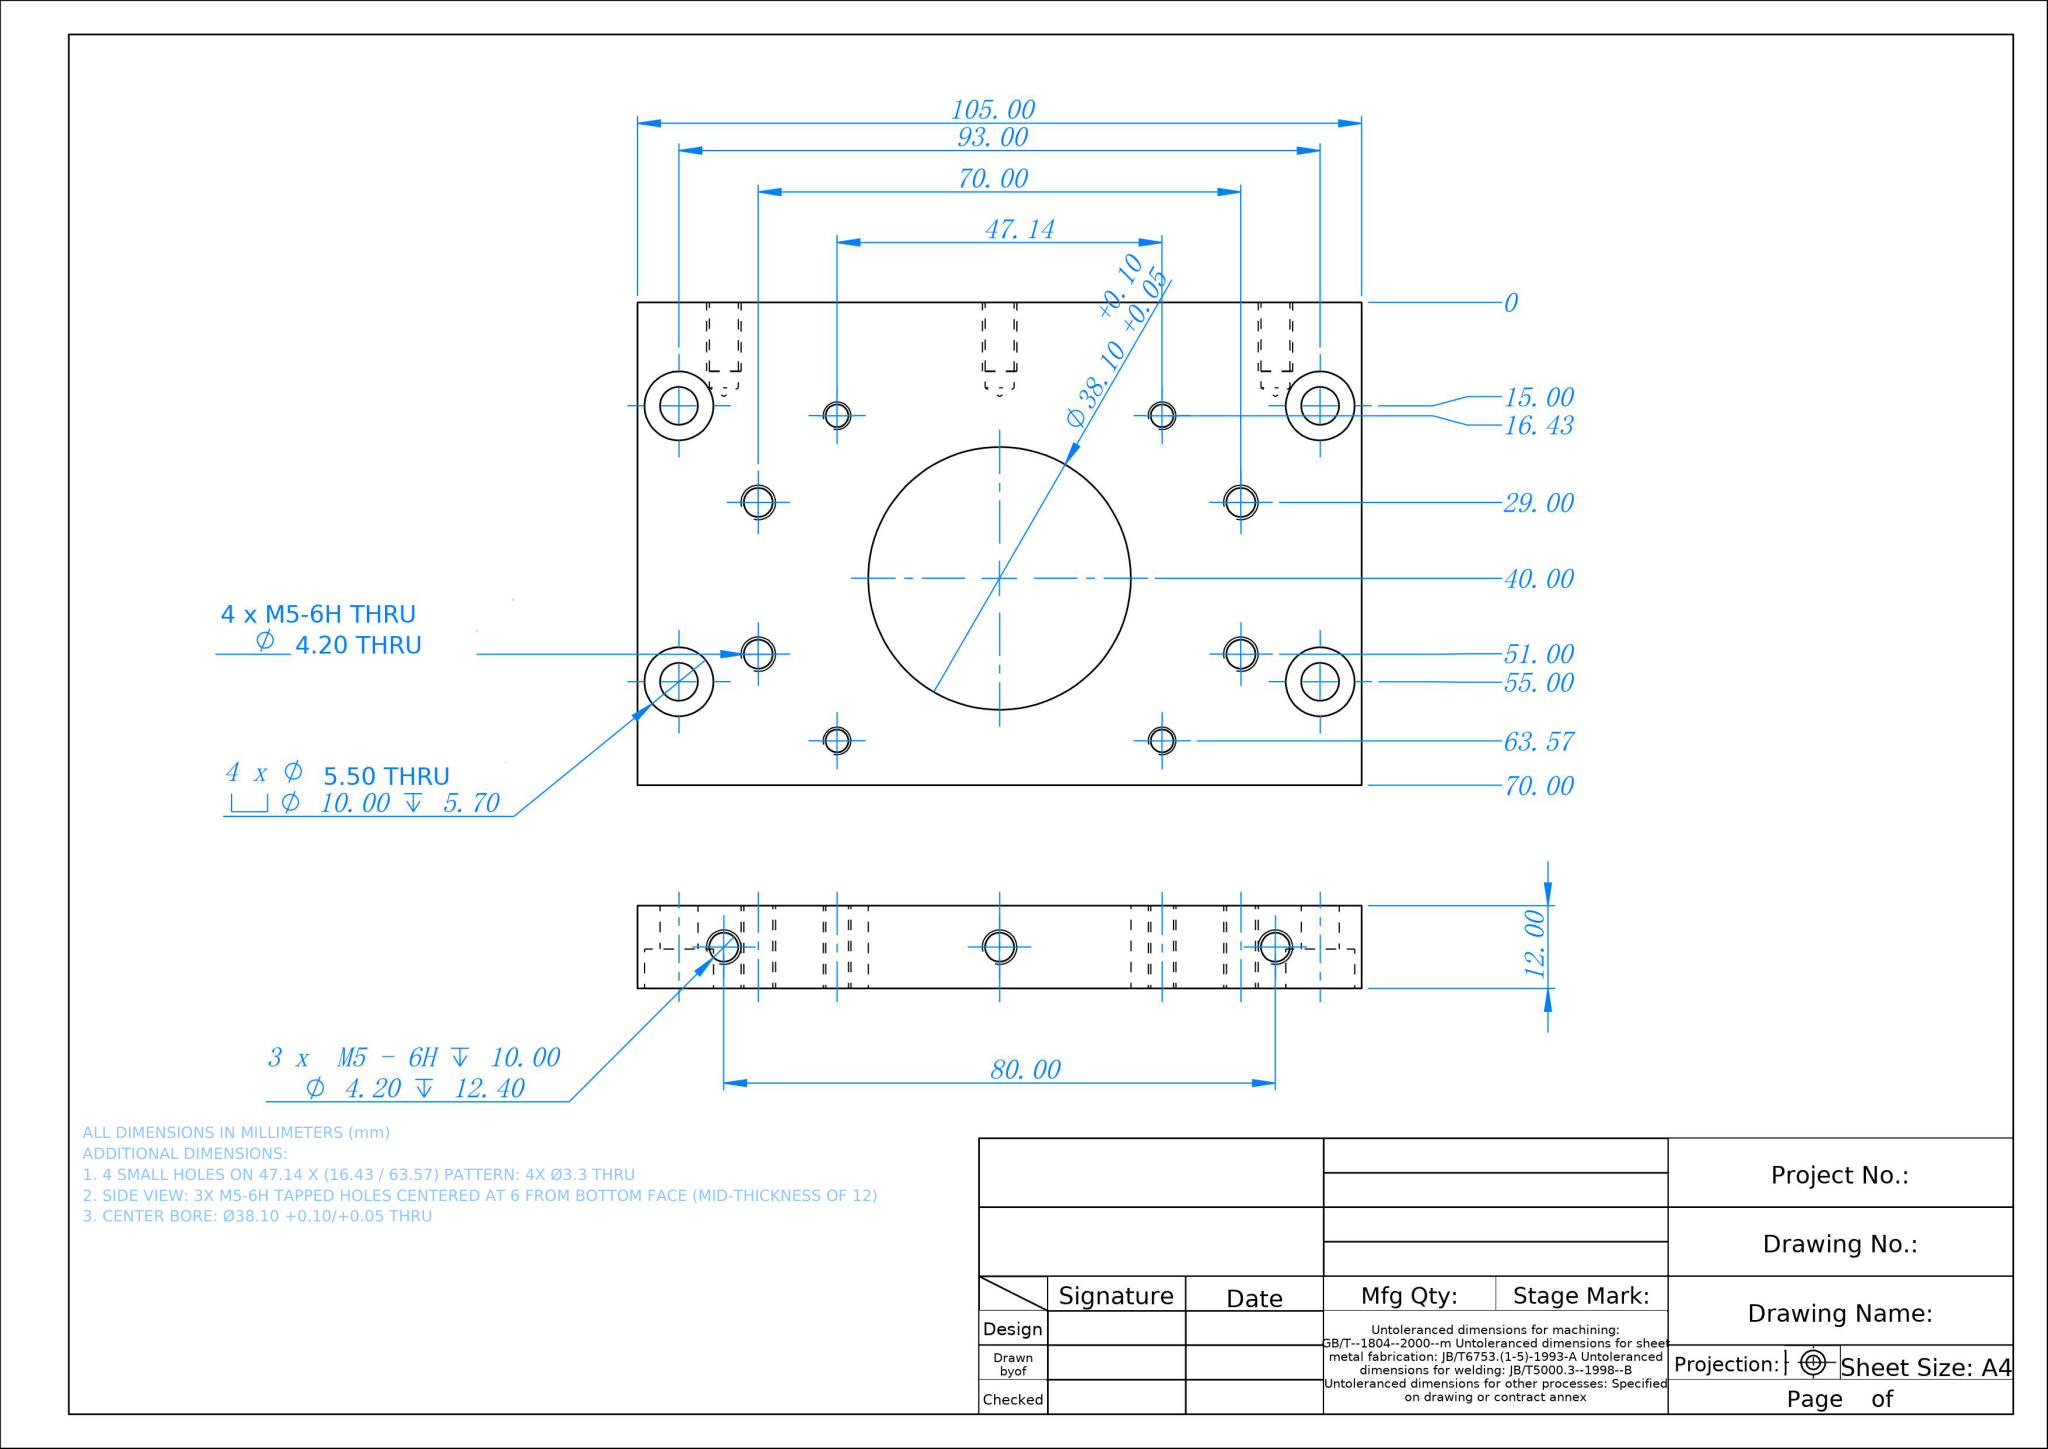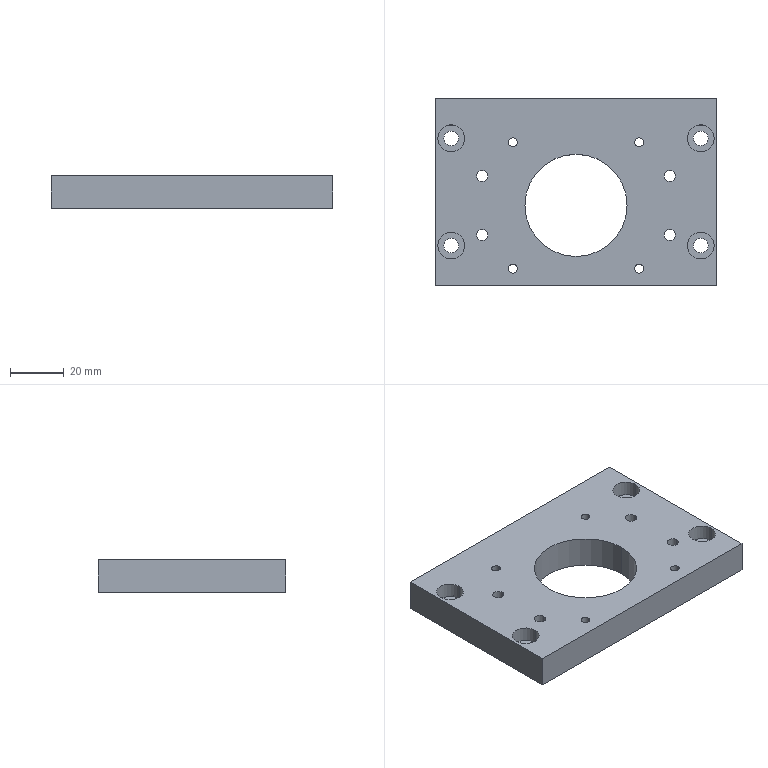Part | NX | mm | 1 solid | 56 faces | box 105 x 70 x 12 mm | volume 70521 mm3 | cylinder 40 | plane 10 | cone 6 | commonest cylinder face diameters 4.2 x14 10 x8 5.5 x8 3.3 x8 38.1 x2